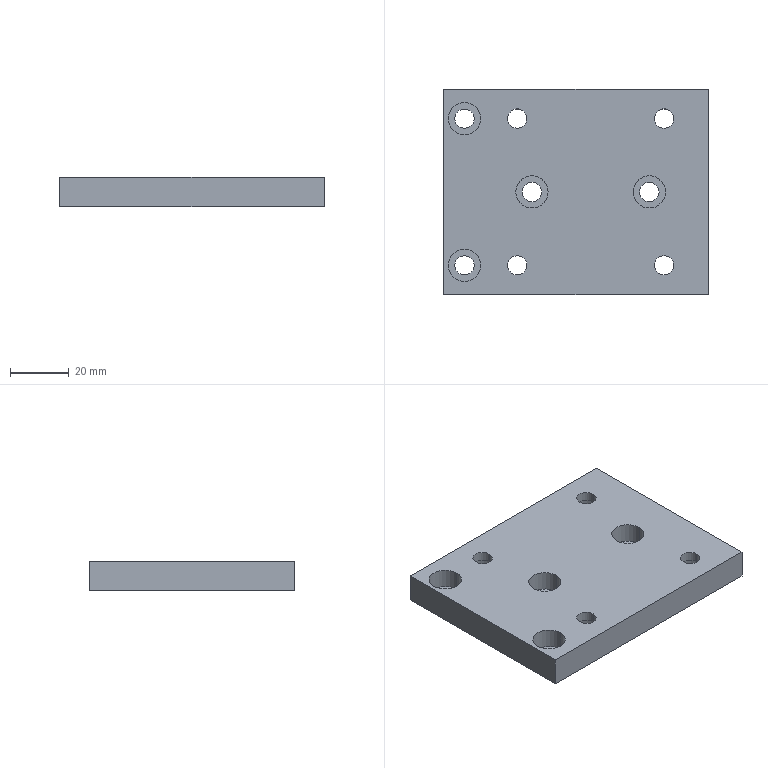Component | SolidWorks | 01-04MarkingMachineMountingBasePlate-1 | 1 solid | 46 faces | box 90 x 70 x 10 mm | volume 56954 mm3 | cylinder 32 | plane 14 | commonest cylinder face diameters 11 x16 6.6 x16 | material A3 Steel
build123d program:
from build123d import *

# Parameters (mm, degrees)
SKETCH1_W                                          = 90
SKETCH1_H                                          = 70
BOSS_EXTRUDE1_DEPTH                                = 5
HOLE_SIZE_ACCORDING_TO_TYPE_1_OF_HEXAG_D           = 6.6
HOLE_SIZE_ACCORDING_TO_TYPE_1_OF_HEXAG_CBORE_D     = 11
HOLE_SIZE_ACCORDING_TO_TYPE_1_OF_HEXAG_CBORE_DEPTH = 6.8
HOLE_SIZE_ACCORDING_TO_TYPE_2_OF_HEXAG_D           = 6.6
HOLE_SIZE_ACCORDING_TO_TYPE_2_OF_HEXAG_CBORE_D     = 11
HOLE_SIZE_ACCORDING_TO_TYPE_2_OF_HEXAG_CBORE_DEPTH = 6.8
HOLE_SIZE_ACCORDING_TO_TYPE_3_OF_HEXAG_D           = 6.6
HOLE_SIZE_ACCORDING_TO_TYPE_3_OF_HEXAG_CBORE_D     = 11
HOLE_SIZE_ACCORDING_TO_TYPE_3_OF_HEXAG_CBORE_DEPTH = 6.8


with BuildPart() as part:
    # Sketch1 → Boss-Extrude1 (new, symmetric)
    with BuildSketch(Plane.XY):
        Rectangle(SKETCH1_W, SKETCH1_H)
    extrude(amount=BOSS_EXTRUDE1_DEPTH, both=True)

    # Hole Size _According to_ Type 1 of Hexag (through all)
    with Locations(Plane(origin=(-38, 25, 5), x_dir=(1, 0, 0), z_dir=(0, 0, 1))):
        with Locations((0, 0), (0, -50)):
            CounterBoreHole(HOLE_SIZE_ACCORDING_TO_TYPE_1_OF_HEXAG_D / 2, HOLE_SIZE_ACCORDING_TO_TYPE_1_OF_HEXAG_CBORE_D / 2, HOLE_SIZE_ACCORDING_TO_TYPE_1_OF_HEXAG_CBORE_DEPTH)

    # Hole Size _According to_ Type 2 of Hexag (through all)
    with Locations(Plane(origin=(30, 25, -5), x_dir=(-1, 0, 0), z_dir=(0, 0, -1))):
        with Locations((0, 0), (50, 0), (50, -50), (0, -50)):
            CounterBoreHole(HOLE_SIZE_ACCORDING_TO_TYPE_2_OF_HEXAG_D / 2, HOLE_SIZE_ACCORDING_TO_TYPE_2_OF_HEXAG_CBORE_D / 2, HOLE_SIZE_ACCORDING_TO_TYPE_2_OF_HEXAG_CBORE_DEPTH)

    # Hole Size _According to_ Type 3 of Hexag (through all)
    with Locations(Plane(origin=(-15, 0, 5), x_dir=(1, 0, 0), z_dir=(0, 0, 1))):
        with Locations((0, 0), (40, 0)):
            CounterBoreHole(HOLE_SIZE_ACCORDING_TO_TYPE_3_OF_HEXAG_D / 2, HOLE_SIZE_ACCORDING_TO_TYPE_3_OF_HEXAG_CBORE_D / 2, HOLE_SIZE_ACCORDING_TO_TYPE_3_OF_HEXAG_CBORE_DEPTH)


solid = part.part

# Placed as in the assembly
solid = solid.moved(Location((-13.91, 2.41, 90), (0, 0, 0)))